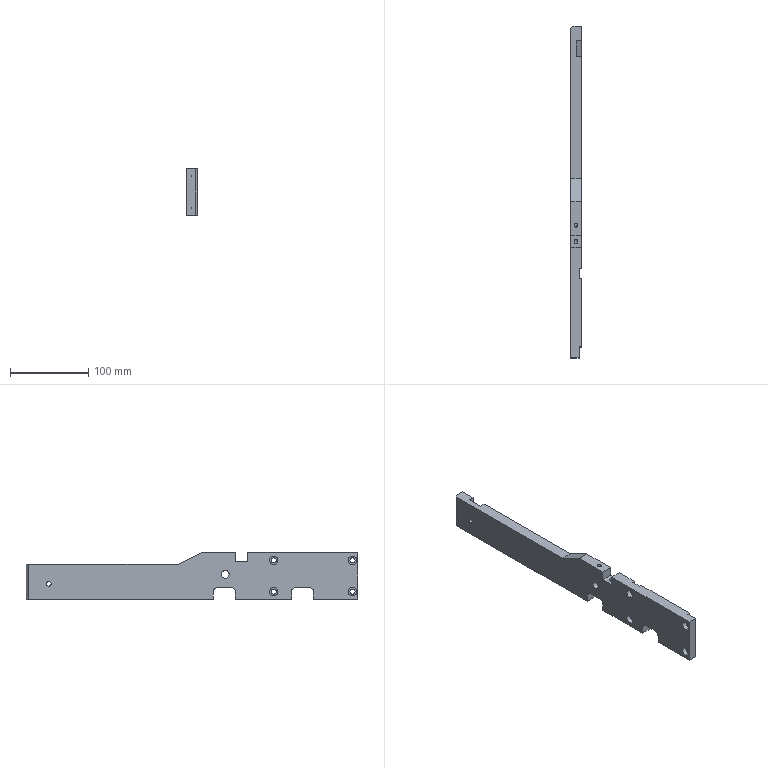Component | SolidWorks | OPW-05-002-1 | 1 solid | 80 faces | box 14 x 425 x 60 mm | volume 285885 mm3 | cylinder 36 | plane 34 | cone 10 | commonest cylinder face diameters 5 x12 11 x8 6.6 x8 10 x6 6 x2
build123d program:
from build123d import *

# Parameters (mm, degrees)
SKETCH1_W                                       = 60
SKETCH1_H                                       = 425
BOSS_EXTRUDE1_DEPTH                             = 7
SKETCH2_W                                       = 60
SKETCH2_H                                       = 14
SKETCH2_H_2                                     = 12
CUT_EXTRUDE1_DEPTH                              = 3
M6_HEX_SOCKET_HEAD_CAP_SCREW_CBORE1_D           = 6.6
M6_HEX_SOCKET_HEAD_CAP_SCREW_CBORE1_CBORE_D     = 11
M6_HEX_SOCKET_HEAD_CAP_SCREW_CBORE1_CBORE_DEPTH = 6
M6_TAPPED_HOLE1_D                               = 5
M6_TAPPED_HOLE1_DEPTH                           = 17
M6_TAPPED_HOLE1_TIP                             = 1.502
CUT_EXTRUDE2_REACH                              = 217.063
SKETCH7_W                                       = 15
SKETCH7_H                                       = 28
FILLET1_R                                       = 5
CUT_EXTRUDE3_REACH                              = 217.063
SKETCH8_R                                       = 5
M6_TAPPED_HOLE2_REACH                           = 222.919
M6_TAPPED_HOLE2_BORE_R                          = 2.5
CUT_EXTRUDE4_REACH                              = 217.063
CUT_EXTRUDE5_REACH                              = 217.063
SKETCH12_R                                      = 3
CUT_EXTRUDE6_DEPTH                              = 10
CHAMFER2_SIZE                                   = 3
SKETCH14_W                                      = 14
SKETCH14_H                                      = 16
CUT_EXTRUDE7_DEPTH                              = 12
M6_TAPPED_HOLE3_D                               = 5
M6_TAPPED_HOLE3_DEPTH                           = 17
M6_TAPPED_HOLE3_TIP                             = 1.502
M6_TAPPED_HOLE4_D                               = 5
M6_TAPPED_HOLE4_DEPTH                           = 15
M6_TAPPED_HOLE4_TIP                             = 1.502


with BuildPart() as part:
    # Sketch1 → Boss-Extrude1 (new, symmetric)
    with BuildSketch(Plane.XY):
        Rectangle(SKETCH1_W, SKETCH1_H)
    extrude(amount=BOSS_EXTRUDE1_DEPTH, both=True)

    # Sketch2 → Cut-Extrude1 (cut)
    with BuildSketch(Plane(origin=(0, 0, -7), x_dir=(-1, 0, 0), z_dir=(0, 0, -1))):
        with Locations((0, -205.5)):
            Rectangle(SKETCH2_W, SKETCH2_H)
        with Locations((0, -104.5)):
            Rectangle(SKETCH2_W, SKETCH2_H_2)
    extrude(amount=-CUT_EXTRUDE1_DEPTH, mode=Mode.SUBTRACT)

    # M6 Hex Socket Head Cap Screw CBORE1 (through all)
    with Locations(Plane.XY.offset(7)):
        with Locations((-20, -205.5), (20, -205.5), (20, -104.5), (-20, -104.5)):
            CounterBoreHole(M6_HEX_SOCKET_HEAD_CAP_SCREW_CBORE1_D / 2, M6_HEX_SOCKET_HEAD_CAP_SCREW_CBORE1_CBORE_D / 2, M6_HEX_SOCKET_HEAD_CAP_SCREW_CBORE1_CBORE_DEPTH)

    # M6 Tapped Hole1
    with Locations(Plane.ZY.offset(30)):
        with Locations((0, -181.5), (0, -163.5)):
            Hole(M6_TAPPED_HOLE1_D / 2, depth=M6_TAPPED_HOLE1_DEPTH)
            with Locations((0, 0, -(M6_TAPPED_HOLE1_DEPTH + M6_TAPPED_HOLE1_TIP / 2))):  # 118° drill point
                Cone(0, M6_TAPPED_HOLE1_D / 2, M6_TAPPED_HOLE1_TIP, mode=Mode.SUBTRACT)

    # Sketch7 → Cut-Extrude2 (cut, up to next)
    with BuildSketch(Plane.XY.offset(7), mode=Mode.PRIVATE) as cut_extrude2_sk1:
        with Locations((-22.5, -141.5)):
            Rectangle(SKETCH7_W, SKETCH7_H)
    cut_extrude2_tool1 = extrude(cut_extrude2_sk1.sketch, amount=-CUT_EXTRUDE2_REACH, mode=Mode.PRIVATE) & part.part
    # Sketch7 → Cut-Extrude2 (cut, up to next)
    with BuildSketch(Plane.XY.offset(7), mode=Mode.PRIVATE) as cut_extrude2_sk2:
        with Locations((-22.5, -41.5)):
            Rectangle(SKETCH7_W, SKETCH7_H)
    cut_extrude2_tool2 = extrude(cut_extrude2_sk2.sketch, amount=-CUT_EXTRUDE2_REACH, mode=Mode.PRIVATE) & part.part
    add(cut_extrude2_tool1.solids().sort_by_distance((-22.5, -141.5, 7))[0], mode=Mode.SUBTRACT)
    add(cut_extrude2_tool2.solids().sort_by_distance((-22.5, -41.5, 7))[0], mode=Mode.SUBTRACT)

    # Fillet1
    fillet1_edges = [part.edges().sort_by_distance(p)[0] for p in [
        (-15, -27.5, 0),
        (-15, -55.5, 0),
        (-15, -127.5, 0),
        (-15, -155.5, 0),
    ]]
    fillet(fillet1_edges, radius=FILLET1_R)

    # Sketch8 → Cut-Extrude3 (cut, up to next)
    with BuildSketch(Plane(origin=(0, 0, -7), x_dir=(-1, 0, 0), z_dir=(0, 0, -1)), mode=Mode.PRIVATE) as cut_extrude3_sk1:
        with Locations((-2, -42.5)):
            Circle(SKETCH8_R)
    cut_extrude3_tool1 = extrude(cut_extrude3_sk1.sketch, amount=-CUT_EXTRUDE3_REACH, mode=Mode.PRIVATE) & part.part
    add(cut_extrude3_tool1.solids().sort_by_distance((2, -42.5, -7))[0], mode=Mode.SUBTRACT)

    # M6 Tapped Hole2 bore → M6 Tapped Hole2 (cut, up to next)
    with BuildSketch(Plane(origin=(30, 0, 0), x_dir=(0, 0, -1), z_dir=(1, 0, 0)), mode=Mode.PRIVATE) as m6_tapped_hole2_sk1:
        with Locations((0, -42.5)):
            Circle(M6_TAPPED_HOLE2_BORE_R)
    m6_tapped_hole2_tool1 = extrude(m6_tapped_hole2_sk1.sketch, amount=-M6_TAPPED_HOLE2_REACH, mode=Mode.PRIVATE) & part.part
    add(m6_tapped_hole2_tool1.solids().sort_by_distance((30, -42.5, 0))[0], mode=Mode.SUBTRACT)

    # Sketch11 → Cut-Extrude4 (cut, up to next)
    with BuildSketch(Plane(origin=(0, 0, -7), x_dir=(-1, 0, 0), z_dir=(0, 0, -1)), mode=Mode.PRIVATE) as cut_extrude4_sk1:
        Polygon((-30, 212.5), (-15, 212.5), (-15, 17.5), (-30, -12.5), align=None)
    cut_extrude4_tool1 = extrude(cut_extrude4_sk1.sketch, amount=-CUT_EXTRUDE4_REACH, mode=Mode.PRIVATE) & part.part
    add(cut_extrude4_tool1.solids().sort_by_distance((22.679, 107.321, -7))[0], mode=Mode.SUBTRACT)

    # Sketch12 → Cut-Extrude5 (cut, up to next)
    with BuildSketch(Plane(origin=(0, 0, -7), x_dir=(-1, 0, 0), z_dir=(0, 0, -1)), mode=Mode.PRIVATE) as cut_extrude5_sk1:
        with Locations((10, 183.5)):
            Circle(SKETCH12_R)
    cut_extrude5_tool1 = extrude(cut_extrude5_sk1.sketch, amount=-CUT_EXTRUDE5_REACH, mode=Mode.PRIVATE) & part.part
    add(cut_extrude5_tool1.solids().sort_by_distance((-10, 183.5, -7))[0], mode=Mode.SUBTRACT)

    # Sketch13 → Cut-Extrude6 (cut, symmetric)
    with BuildSketch(Plane(origin=(0, 183.5, 0), x_dir=(-1, 0, 0), z_dir=(0, 1, 0))):
        Polygon((-15, -0.5), (7, -7), (-15, -7), align=None)
    extrude(amount=CUT_EXTRUDE6_DEPTH, both=True, mode=Mode.SUBTRACT)

    # Chamfer2
    chamfer2_edges = [part.edges().sort_by_distance(p)[0] for p in [
        (-7.5, 212.5, 7),
    ]]
    chamfer(chamfer2_edges, length=CHAMFER2_SIZE)

    # Sketch14 → Cut-Extrude7 (cut)
    with BuildSketch(Plane(origin=(30, 0, 0), x_dir=(0, 0, -1), z_dir=(1, 0, 0))):
        with Locations((0, -63.5)):
            Rectangle(SKETCH14_W, SKETCH14_H)
    extrude(amount=-CUT_EXTRUDE7_DEPTH, mode=Mode.SUBTRACT)

    # M6 Tapped Hole3
    with Locations(Plane(origin=(18, 0, 0), x_dir=(0, 0, -1), z_dir=(1, 0, 0))):
        with Locations((0, -63.5)):
            Hole(M6_TAPPED_HOLE3_D / 2, depth=M6_TAPPED_HOLE3_DEPTH)
            with Locations((0, 0, -(M6_TAPPED_HOLE3_DEPTH + M6_TAPPED_HOLE3_TIP / 2))):  # 118° drill point
                Cone(0, M6_TAPPED_HOLE3_D / 2, M6_TAPPED_HOLE3_TIP, mode=Mode.SUBTRACT)

    # M6 Tapped Hole4
    with Locations(Plane.ZY.offset(30)):
        with Locations((0, -112.5), (0, -67.5)):
            Hole(M6_TAPPED_HOLE4_D / 2, depth=M6_TAPPED_HOLE4_DEPTH)
            with Locations((0, 0, -(M6_TAPPED_HOLE4_DEPTH + M6_TAPPED_HOLE4_TIP / 2))):  # 118° drill point
                Cone(0, M6_TAPPED_HOLE4_D / 2, M6_TAPPED_HOLE4_TIP, mode=Mode.SUBTRACT)


solid = part.part

# Placed as in the assembly
solid = solid.moved(Location((-247.904, 254.499, 0), (0, -90, 0)))